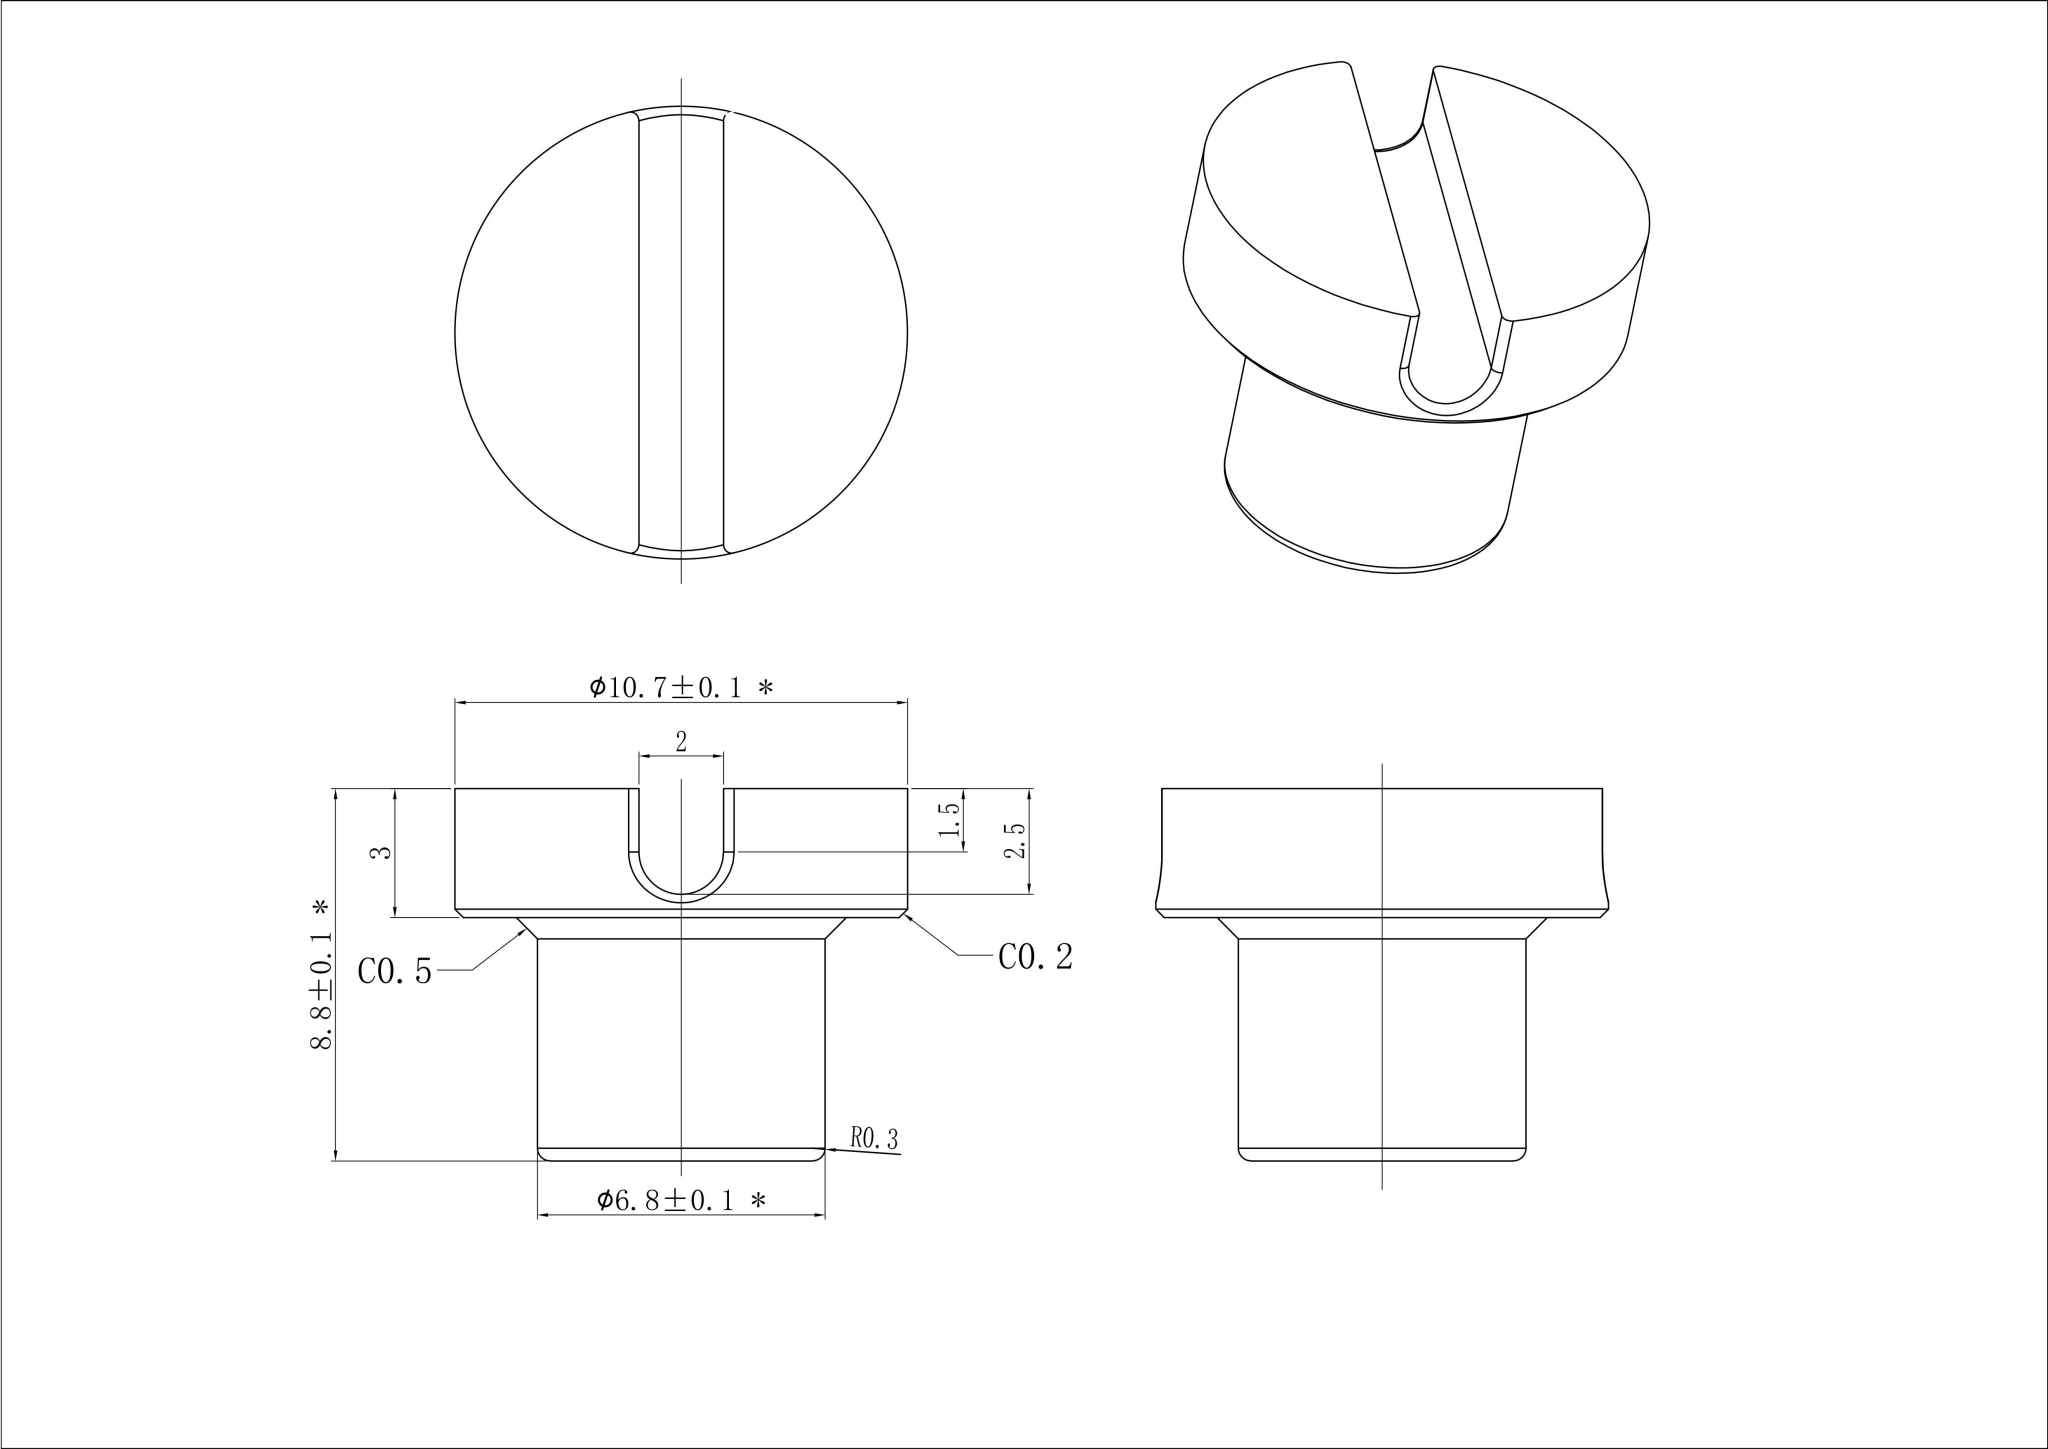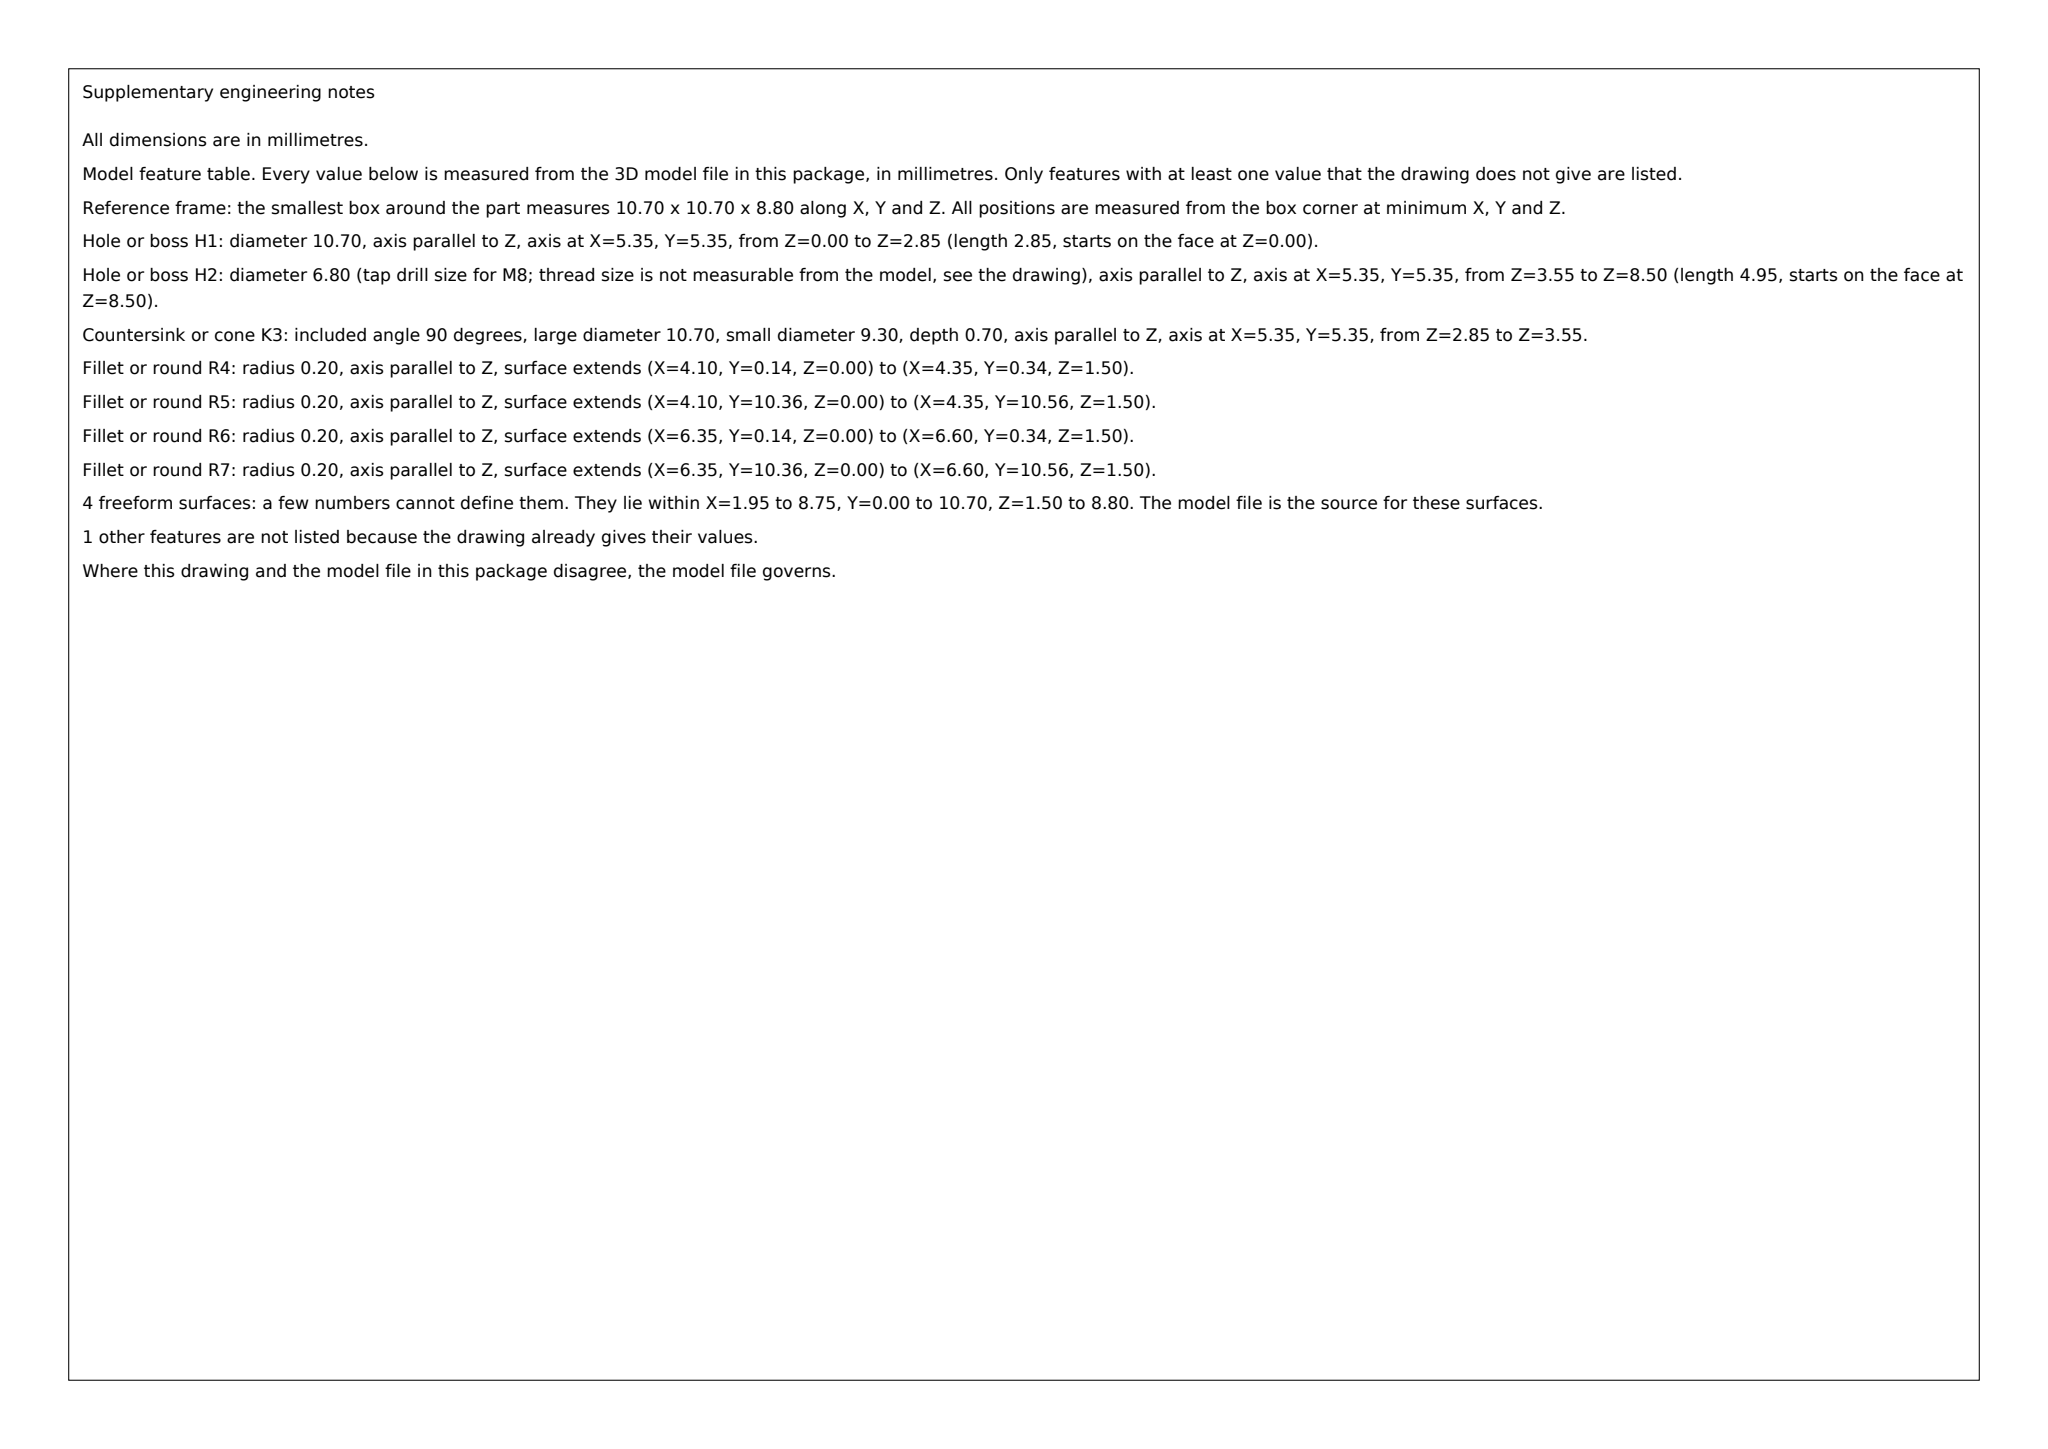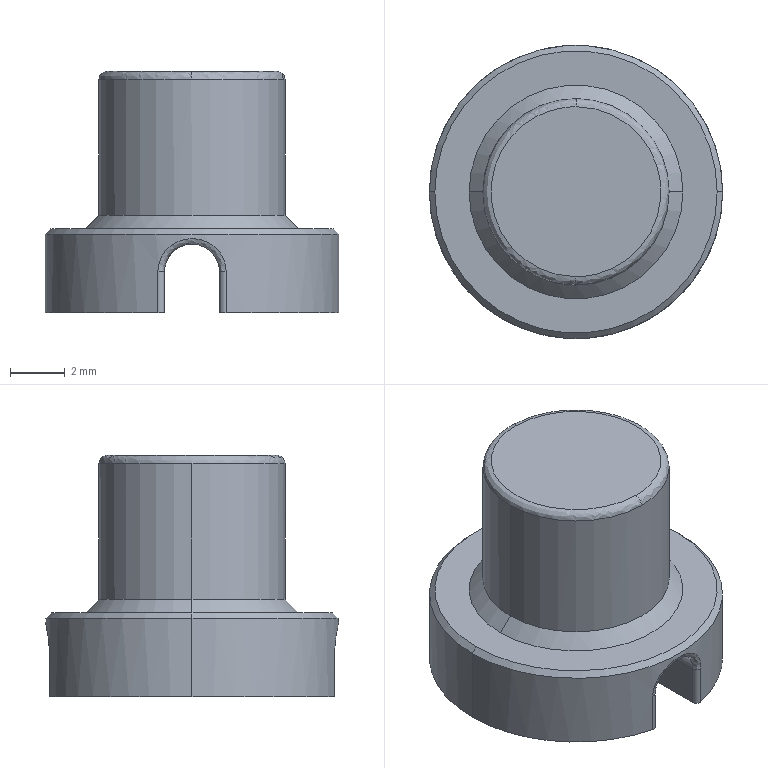Part | SolidWorks | mm | 1 solid | 23 faces | box 10.7 x 10.7 x 8.8 mm | volume 436 mm3 | cylinder 9 | plane 6 | spline 4 | cone 4 | commonest cylinder face diameters 0.4 x4 10.7 x2 6.8 x2 2 x1